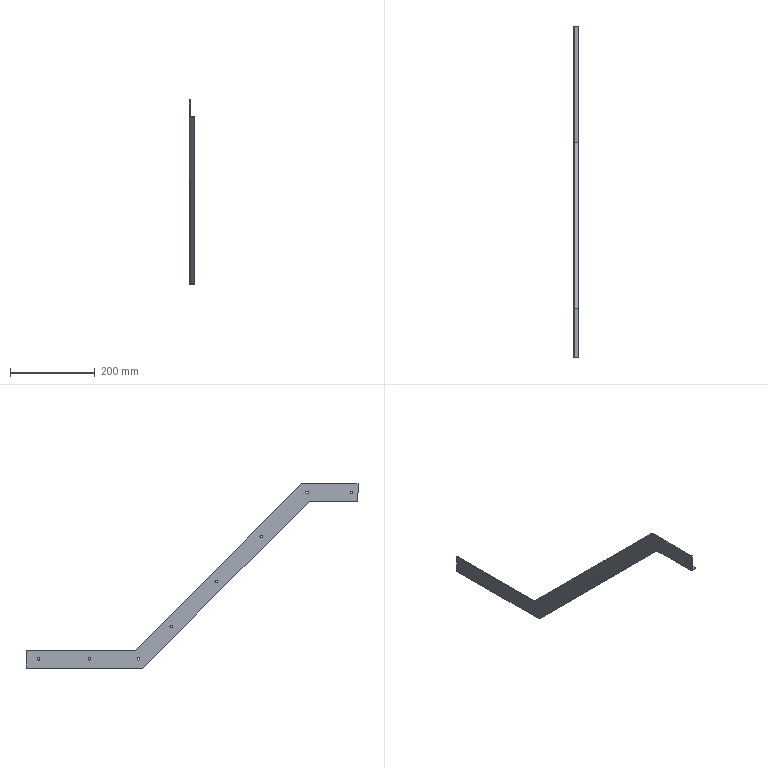Component | SolidWorks | ScraperPlate-1 | 1 solid | 30 faces | box 13 x 782.44 x 434.44 mm | volume 99718 mm3 | cylinder 16 | plane 14 | commonest cylinder face diameters 6 x16
build123d program:
from build123d import *

# Parameters (mm, degrees)
EXTRUDE_THIN1_DEPTH = 13
EXTRUDE_THIN2_DEPTH = 2
SKETCH4_R           = 3
CUT_EXTRUDE1_DEPTH  = 10


with BuildPart() as part:
    # Sketch1 → Extrude-Thin1 (new body)
    with BuildSketch(Plane.XY):
        Polygon((365.38, 490.188), (365.38, 215.188), (-27.064, -177.256), (-27.064, -292.256), (-29.064, -292.256), (-29.064, -176.427), (363.38, 216.017), (363.38, 490.188), align=None)
    extrude(amount=EXTRUDE_THIN1_DEPTH)

    # Sketch2 → Extrude-Thin2 (add)
    with BuildSketch(Plane(origin=(0, 0, 0), x_dir=(-1, 0, 0), z_dir=(0, 0, -1))):
        Polygon((-365.38, 490.188), (-365.38, 215.188), (27.064, -177.256), (27.064, -292.256), (69.064, -292.256), (69.064, -159.859), (-323.38, 232.585), (-323.38, 490.188), align=None)
    extrude(amount=-EXTRUDE_THIN2_DEPTH)

    # Sketch4 → Cut-Extrude1 (cut)
    with BuildSketch(Plane.XY.offset(2)):
        with Locations((343.38, 460.188)):
            Circle(SKETCH4_R)
        with Locations((343.38, 340.188)):
            Circle(SKETCH4_R)
        with Locations((267.057, 147.979)):
            Circle(SKETCH4_R)
        with Locations((160.991, 41.913)):
            Circle(SKETCH4_R)
        with Locations((54.925, -64.153)):
            Circle(SKETCH4_R)
        with Locations((-49.064, -277.256)):
            Circle(SKETCH4_R)
        with Locations((-49.064, -172.256)):
            Circle(SKETCH4_R)
        with Locations((343.38, 225.188)):
            Circle(SKETCH4_R)
    extrude(amount=-CUT_EXTRUDE1_DEPTH, mode=Mode.SUBTRACT)


solid = part.part

# Placed as in the assembly
solid = solid.moved(Location((-292.55, -121.313, -21.856), (0, 90, 0)))
STEP:
#1=CARTESIAN_POINT('',(-11.518,4.09,-14.497));
#2=VERTEX_POINT('',#1);
#3=CARTESIAN_POINT('',(-11.518,4.09,-14.261));
#4=VERTEX_POINT('',#3);
#5=CARTESIAN_POINT('',(-11.518,4.09,-14.379));
#6=DIRECTION('',(-1.,-0.,-0.));
#7=DIRECTION('',(0.,-0.,1.));
#8=AXIS2_PLACEMENT_3D('',#5,#6,#7);
#9=CIRCLE('',#8,0.1181);
#10=EDGE_CURVE('',#2,#4,#9,.T.);
#11=ORIENTED_EDGE('',*,*,#10,.T.);
#12=CARTESIAN_POINT('',(-11.439,4.09,-14.261));
#13=VERTEX_POINT('',#12);
#14=CARTESIAN_POINT('',(-11.833,4.09,-14.261));
#15=DIRECTION('',(1.,0.,0.));
#16=VECTOR('',#15,39.37);
#17=LINE('',#14,#16);
#18=EDGE_CURVE('',#4,#13,#17,.T.);
#19=ORIENTED_EDGE('',*,*,#18,.T.);
#20=CARTESIAN_POINT('',(-11.439,4.09,-14.497));
#21=VERTEX_POINT('',#20);
#22=CARTESIAN_POINT('',(-11.439,4.09,-14.379));
#23=DIRECTION('',(1.,0.,0.));
#24=DIRECTION('',(0.,0.,-1.));
#25=AXIS2_PLACEMENT_3D('',#22,#23,#24);
#26=CIRCLE('',#25,0.1181);
#27=EDGE_CURVE('',#13,#21,#26,.T.);
#28=ORIENTED_EDGE('',*,*,#27,.T.);
#29=CARTESIAN_POINT('',(-11.833,4.09,-14.497));
#30=DIRECTION('',(1.,0.,0.));
#31=VECTOR('',#30,39.37);
#32=LINE('',#29,#31);
#33=EDGE_CURVE('',#2,#21,#32,.T.);
#34=ORIENTED_EDGE('',*,*,#33,.F.);
#35=EDGE_LOOP('',(#11,#19,#28,#34));
#36=FACE_OUTER_BOUND('',#35,.T.);
#37=CARTESIAN_POINT('',(-11.833,4.09,-14.379));
#38=DIRECTION('',(1.,0.,0.));
#39=DIRECTION('',(0.,0.,-1.));
#40=AXIS2_PLACEMENT_3D('',#37,#38,#39);
#41=CYLINDRICAL_SURFACE('',#40,0.1181);
#42=ADVANCED_FACE('',(#36),#41,.F.);
#43=CARTESIAN_POINT('',(-11.518,-11.558,0.9531));
#44=VERTEX_POINT('',#43);
#45=CARTESIAN_POINT('',(-11.518,-11.558,1.189));
#46=VERTEX_POINT('',#45);
#47=CARTESIAN_POINT('',(-11.518,-11.558,1.071));
#48=DIRECTION('',(-1.,-0.,-0.));
#49=DIRECTION('',(0.,0.,1.));
#50=AXIS2_PLACEMENT_3D('',#47,#48,#49);
#51=CIRCLE('',#50,0.1181);
#52=EDGE_CURVE('',#44,#46,#51,.T.);
#53=ORIENTED_EDGE('',*,*,#52,.T.);
#54=CARTESIAN_POINT('',(-11.439,-11.558,1.189));
#55=VERTEX_POINT('',#54);
#56=CARTESIAN_POINT('',(-11.833,-11.558,1.189));
#57=DIRECTION('',(1.,0.,0.));
#58=VECTOR('',#57,39.37);
#59=LINE('',#56,#58);
#60=EDGE_CURVE('',#46,#55,#59,.T.);
#61=ORIENTED_EDGE('',*,*,#60,.T.);
#62=CARTESIAN_POINT('',(-11.439,-11.558,0.9531));
#63=VERTEX_POINT('',#62);
#64=CARTESIAN_POINT('',(-11.439,-11.558,1.071));
#65=DIRECTION('',(1.,0.,0.));
#66=DIRECTION('',(0.,0.,-1.));
#67=AXIS2_PLACEMENT_3D('',#64,#65,#66);
#68=CIRCLE('',#67,0.1181);
#69=EDGE_CURVE('',#55,#63,#68,.T.);
#70=ORIENTED_EDGE('',*,*,#69,.T.);
#71=CARTESIAN_POINT('',(-11.833,-11.558,0.9531));
#72=DIRECTION('',(1.,0.,0.));
#73=VECTOR('',#72,39.37);
#74=LINE('',#71,#73);
#75=EDGE_CURVE('',#44,#63,#74,.T.);
#76=ORIENTED_EDGE('',*,*,#75,.F.);
#77=EDGE_LOOP('',(#53,#61,#70,#76));
#78=FACE_OUTER_BOUND('',#77,.T.);
#79=CARTESIAN_POINT('',(-11.833,-11.558,1.071));
#80=DIRECTION('',(1.,0.,0.));
#81=DIRECTION('',(0.,0.,-1.));
#82=AXIS2_PLACEMENT_3D('',#79,#80,#81);
#83=CYLINDRICAL_SURFACE('',#82,0.1181);
#84=ADVANCED_FACE('',(#78),#83,.F.);
#85=CARTESIAN_POINT('',(-11.518,-15.692,0.9531));
#86=VERTEX_POINT('',#85);
#87=CARTESIAN_POINT('',(-11.518,-15.692,1.189));
#88=VERTEX_POINT('',#87);
#89=CARTESIAN_POINT('',(-11.518,-15.692,1.071));
#90=DIRECTION('',(-1.,-0.,-0.));
#91=DIRECTION('',(0.,0.,1.));
#92=AXIS2_PLACEMENT_3D('',#89,#90,#91);
#93=CIRCLE('',#92,0.1181);
#94=EDGE_CURVE('',#86,#88,#93,.T.);
#95=ORIENTED_EDGE('',*,*,#94,.T.);
#96=CARTESIAN_POINT('',(-11.439,-15.692,1.189));
#97=VERTEX_POINT('',#96);
#98=CARTESIAN_POINT('',(-11.833,-15.692,1.189));
#99=DIRECTION('',(1.,0.,0.));
#100=VECTOR('',#99,39.37);
#101=LINE('',#98,#100);
#102=EDGE_CURVE('',#88,#97,#101,.T.);
#103=ORIENTED_EDGE('',*,*,#102,.T.);
#104=CARTESIAN_POINT('',(-11.439,-15.692,0.9531));
#105=VERTEX_POINT('',#104);
#106=CARTESIAN_POINT('',(-11.439,-15.692,1.071));
#107=DIRECTION('',(1.,0.,0.));
#108=DIRECTION('',(0.,0.,-1.));
#109=AXIS2_PLACEMENT_3D('',#106,#107,#108);
#110=CIRCLE('',#109,0.1181);
#111=EDGE_CURVE('',#97,#105,#110,.T.);
#112=ORIENTED_EDGE('',*,*,#111,.T.);
#113=CARTESIAN_POINT('',(-11.833,-15.692,0.9531));
#114=DIRECTION('',(1.,0.,0.));
#115=VECTOR('',#114,39.37);
#116=LINE('',#113,#115);
#117=EDGE_CURVE('',#86,#105,#116,.T.);
#118=ORIENTED_EDGE('',*,*,#117,.F.);
#119=EDGE_LOOP('',(#95,#103,#112,#118));
#120=FACE_OUTER_BOUND('',#119,.T.);
#121=CARTESIAN_POINT('',(-11.833,-15.692,1.071));
#122=DIRECTION('',(1.,0.,0.));
#123=DIRECTION('',(0.,0.,-1.));
#124=AXIS2_PLACEMENT_3D('',#121,#122,#123);
#125=CYLINDRICAL_SURFACE('',#124,0.1181);
#126=ADVANCED_FACE('',(#120),#125,.F.);
#127=CARTESIAN_POINT('',(-11.518,-7.302,-3.141));
#128=VERTEX_POINT('',#127);
#129=CARTESIAN_POINT('',(-11.518,-7.302,-2.905));
#130=VERTEX_POINT('',#129);
#131=CARTESIAN_POINT('',(-11.518,-7.302,-3.023));
#132=DIRECTION('',(-1.,-0.,-0.));
#133=DIRECTION('',(0.,0.,1.));
#134=AXIS2_PLACEMENT_3D('',#131,#132,#133);
#135=CIRCLE('',#134,0.1181);
#136=EDGE_CURVE('',#128,#130,#135,.T.);
#137=ORIENTED_EDGE('',*,*,#136,.T.);
#138=CARTESIAN_POINT('',(-11.439,-7.302,-2.905));
#139=VERTEX_POINT('',#138);
#140=CARTESIAN_POINT('',(-11.833,-7.302,-2.905));
#141=DIRECTION('',(1.,0.,0.));
#142=VECTOR('',#141,39.37);
#143=LINE('',#140,#142);
#144=EDGE_CURVE('',#130,#139,#143,.T.);
#145=ORIENTED_EDGE('',*,*,#144,.T.);
#146=CARTESIAN_POINT('',(-11.439,-7.302,-3.141));
#147=VERTEX_POINT('',#146);
#148=CARTESIAN_POINT('',(-11.439,-7.302,-3.023));
#149=DIRECTION('',(1.,0.,0.));
#150=DIRECTION('',(0.,0.,-1.));
#151=AXIS2_PLACEMENT_3D('',#148,#149,#150);
#152=CIRCLE('',#151,0.1181);
#153=EDGE_CURVE('',#139,#147,#152,.T.);
#154=ORIENTED_EDGE('',*,*,#153,.T.);
#155=CARTESIAN_POINT('',(-11.833,-7.302,-3.141));
#156=DIRECTION('',(1.,0.,0.));
#157=VECTOR('',#156,39.37);
#158=LINE('',#155,#157);
#159=EDGE_CURVE('',#128,#147,#158,.T.);
#160=ORIENTED_EDGE('',*,*,#159,.F.);
#161=EDGE_LOOP('',(#137,#145,#154,#160));
#162=FACE_OUTER_BOUND('',#161,.T.);
#163=CARTESIAN_POINT('',(-11.833,-7.302,-3.023));
#164=DIRECTION('',(1.,0.,0.));
#165=DIRECTION('',(0.,0.,-1.));
#166=AXIS2_PLACEMENT_3D('',#163,#164,#165);
#167=CYLINDRICAL_SURFACE('',#166,0.1181);
#168=ADVANCED_FACE('',(#162),#167,.F.);
#169=CARTESIAN_POINT('',(-11.518,-3.126,-7.317));
#170=VERTEX_POINT('',#169);
#171=CARTESIAN_POINT('',(-11.518,-3.126,-7.081));
#172=VERTEX_POINT('',#171);
#173=CARTESIAN_POINT('',(-11.518,-3.126,-7.199));
#174=DIRECTION('',(-1.,-0.,-0.));
#175=DIRECTION('',(0.,-0.,1.));
#176=AXIS2_PLACEMENT_3D('',#173,#174,#175);
#177=CIRCLE('',#176,0.1181);
#178=EDGE_CURVE('',#170,#172,#177,.T.);
#179=ORIENTED_EDGE('',*,*,#178,.T.);
#180=CARTESIAN_POINT('',(-11.439,-3.126,-7.081));
#181=VERTEX_POINT('',#180);
#182=CARTESIAN_POINT('',(-11.833,-3.126,-7.081));
#183=DIRECTION('',(1.,0.,0.));
#184=VECTOR('',#183,39.37);
#185=LINE('',#182,#184);
#186=EDGE_CURVE('',#172,#181,#185,.T.);
#187=ORIENTED_EDGE('',*,*,#186,.T.);
#188=CARTESIAN_POINT('',(-11.439,-3.126,-7.317));
#189=VERTEX_POINT('',#188);
#190=CARTESIAN_POINT('',(-11.439,-3.126,-7.199));
#191=DIRECTION('',(1.,0.,0.));
#192=DIRECTION('',(0.,0.,-1.));
#193=AXIS2_PLACEMENT_3D('',#190,#191,#192);
#194=CIRCLE('',#193,0.1181);
#195=EDGE_CURVE('',#181,#189,#194,.T.);
#196=ORIENTED_EDGE('',*,*,#195,.T.);
#197=CARTESIAN_POINT('',(-11.833,-3.126,-7.317));
#198=DIRECTION('',(1.,0.,0.));
#199=VECTOR('',#198,39.37);
#200=LINE('',#197,#199);
#201=EDGE_CURVE('',#170,#189,#200,.T.);
#202=ORIENTED_EDGE('',*,*,#201,.F.);
#203=EDGE_LOOP('',(#179,#187,#196,#202));
#204=FACE_OUTER_BOUND('',#203,.T.);
#205=CARTESIAN_POINT('',(-11.833,-3.126,-7.199));
#206=DIRECTION('',(1.,0.,0.));
#207=DIRECTION('',(0.,0.,-1.));
#208=AXIS2_PLACEMENT_3D('',#205,#206,#207);
#209=CYLINDRICAL_SURFACE('',#208,0.1181);
#210=ADVANCED_FACE('',(#204),#209,.F.);
#211=CARTESIAN_POINT('',(-11.518,1.05,-11.493));
#212=VERTEX_POINT('',#211);
#213=CARTESIAN_POINT('',(-11.518,1.05,-11.256));
#214=VERTEX_POINT('',#213);
#215=CARTESIAN_POINT('',(-11.518,1.05,-11.375));
#216=DIRECTION('',(-1.,-0.,-0.));
#217=DIRECTION('',(0.,-0.,1.));
#218=AXIS2_PLACEMENT_3D('',#215,#216,#217);
#219=CIRCLE('',#218,0.1181);
#220=EDGE_CURVE('',#212,#214,#219,.T.);
#221=ORIENTED_EDGE('',*,*,#220,.T.);
#222=CARTESIAN_POINT('',(-11.439,1.05,-11.256));
#223=VERTEX_POINT('',#222);
#224=CARTESIAN_POINT('',(-11.833,1.05,-11.256));
#225=DIRECTION('',(1.,0.,0.));
#226=VECTOR('',#225,39.37);
#227=LINE('',#224,#226);
#228=EDGE_CURVE('',#214,#223,#227,.T.);
#229=ORIENTED_EDGE('',*,*,#228,.T.);
#230=CARTESIAN_POINT('',(-11.439,1.05,-11.493));
#231=VERTEX_POINT('',#230);
#232=CARTESIAN_POINT('',(-11.439,1.05,-11.375));
#233=DIRECTION('',(1.,0.,0.));
#234=DIRECTION('',(0.,0.,-1.));
#235=AXIS2_PLACEMENT_3D('',#232,#233,#234);
#236=CIRCLE('',#235,0.1181);
#237=EDGE_CURVE('',#223,#231,#236,.T.);
#238=ORIENTED_EDGE('',*,*,#237,.T.);
#239=CARTESIAN_POINT('',(-11.833,1.05,-11.493));
#240=DIRECTION('',(1.,0.,0.));
#241=VECTOR('',#240,39.37);
#242=LINE('',#239,#241);
#243=EDGE_CURVE('',#212,#231,#242,.T.);
#244=ORIENTED_EDGE('',*,*,#243,.F.);
#245=EDGE_LOOP('',(#221,#229,#238,#244));
#246=FACE_OUTER_BOUND('',#245,.T.);
#247=CARTESIAN_POINT('',(-11.833,1.05,-11.375));
#248=DIRECTION('',(1.,0.,0.));
#249=DIRECTION('',(0.,0.,-1.));
#250=AXIS2_PLACEMENT_3D('',#247,#248,#249);
#251=CYLINDRICAL_SURFACE('',#250,0.1181);
#252=ADVANCED_FACE('',(#246),#251,.F.);
#253=CARTESIAN_POINT('',(-11.518,8.617,-14.497));
#254=VERTEX_POINT('',#253);
#255=CARTESIAN_POINT('',(-11.518,8.617,-14.261));
#256=VERTEX_POINT('',#255);
#257=CARTESIAN_POINT('',(-11.518,8.617,-14.379));
#258=DIRECTION('',(-1.,-0.,-0.));
#259=DIRECTION('',(0.,0.,1.));
#260=AXIS2_PLACEMENT_3D('',#257,#258,#259);
#261=CIRCLE('',#260,0.1181);
#262=EDGE_CURVE('',#254,#256,#261,.T.);
#263=ORIENTED_EDGE('',*,*,#262,.T.);
#264=CARTESIAN_POINT('',(-11.439,8.617,-14.261));
#265=VERTEX_POINT('',#264);
#266=CARTESIAN_POINT('',(-11.833,8.617,-14.261));
#267=DIRECTION('',(1.,0.,0.));
#268=VECTOR('',#267,39.37);
#269=LINE('',#266,#268);
#270=EDGE_CURVE('',#256,#265,#269,.T.);
#271=ORIENTED_EDGE('',*,*,#270,.T.);
#272=CARTESIAN_POINT('',(-11.439,8.617,-14.497));
#273=VERTEX_POINT('',#272);
#274=CARTESIAN_POINT('',(-11.439,8.617,-14.379));
#275=DIRECTION('',(1.,0.,0.));
#276=DIRECTION('',(0.,0.,-1.));
#277=AXIS2_PLACEMENT_3D('',#274,#275,#276);
#278=CIRCLE('',#277,0.1181);
#279=EDGE_CURVE('',#265,#273,#278,.T.);
#280=ORIENTED_EDGE('',*,*,#279,.T.);
#281=CARTESIAN_POINT('',(-11.833,8.617,-14.497));
#282=DIRECTION('',(1.,0.,0.));
#283=VECTOR('',#282,39.37);
#284=LINE('',#281,#283);
#285=EDGE_CURVE('',#254,#273,#284,.T.);
#286=ORIENTED_EDGE('',*,*,#285,.F.);
#287=EDGE_LOOP('',(#263,#271,#280,#286));
#288=FACE_OUTER_BOUND('',#287,.T.);
#289=CARTESIAN_POINT('',(-11.833,8.617,-14.379));
#290=DIRECTION('',(1.,0.,0.));
#291=DIRECTION('',(0.,0.,-1.));
#292=AXIS2_PLACEMENT_3D('',#289,#290,#291);
#293=CYLINDRICAL_SURFACE('',#292,0.1181);
#294=ADVANCED_FACE('',(#288),#293,.F.);
#295=CARTESIAN_POINT('',(-11.518,13.342,-14.497));
#296=VERTEX_POINT('',#295);
#297=CARTESIAN_POINT('',(-11.518,13.342,-14.261));
#298=VERTEX_POINT('',#297);
#299=CARTESIAN_POINT('',(-11.518,13.342,-14.379));
#300=DIRECTION('',(-1.,-0.,-0.));
#301=DIRECTION('',(0.,0.,1.));
#302=AXIS2_PLACEMENT_3D('',#299,#300,#301);
#303=CIRCLE('',#302,0.1181);
#304=EDGE_CURVE('',#296,#298,#303,.T.);
#305=ORIENTED_EDGE('',*,*,#304,.T.);
#306=CARTESIAN_POINT('',(-11.439,13.342,-14.261));
#307=VERTEX_POINT('',#306);
#308=CARTESIAN_POINT('',(-11.833,13.342,-14.261));
#309=DIRECTION('',(1.,0.,0.));
#310=VECTOR('',#309,39.37);
#311=LINE('',#308,#310);
#312=EDGE_CURVE('',#298,#307,#311,.T.);
#313=ORIENTED_EDGE('',*,*,#312,.T.);
#314=CARTESIAN_POINT('',(-11.439,13.342,-14.497));
#315=VERTEX_POINT('',#314);
#316=CARTESIAN_POINT('',(-11.439,13.342,-14.379));
#317=DIRECTION('',(1.,0.,0.));
#318=DIRECTION('',(0.,0.,-1.));
#319=AXIS2_PLACEMENT_3D('',#316,#317,#318);
#320=CIRCLE('',#319,0.1181);
#321=EDGE_CURVE('',#307,#315,#320,.T.);
#322=ORIENTED_EDGE('',*,*,#321,.T.);
#323=CARTESIAN_POINT('',(-11.833,13.342,-14.497));
#324=DIRECTION('',(1.,0.,0.));
#325=VECTOR('',#324,39.37);
#326=LINE('',#323,#325);
#327=EDGE_CURVE('',#296,#315,#326,.T.);
#328=ORIENTED_EDGE('',*,*,#327,.F.);
#329=EDGE_LOOP('',(#305,#313,#322,#328));
#330=FACE_OUTER_BOUND('',#329,.T.);
#331=CARTESIAN_POINT('',(-11.833,13.342,-14.379));
#332=DIRECTION('',(1.,0.,0.));
#333=DIRECTION('',(0.,0.,-1.));
#334=AXIS2_PLACEMENT_3D('',#331,#332,#333);
#335=CYLINDRICAL_SURFACE('',#334,0.1181);
#336=ADVANCED_FACE('',(#330),#335,.F.);
#337=CARTESIAN_POINT('',(-11.006,-11.722,0.2838));
#338=VERTEX_POINT('',#337);
#339=CARTESIAN_POINT('',(-11.439,-11.722,0.2838));
#340=VERTEX_POINT('',#339);
#341=CARTESIAN_POINT('',(-11.006,-11.722,0.2838));
#342=DIRECTION('',(-1.,-0.,-0.));
#343=VECTOR('',#342,39.37);
#344=LINE('',#341,#343);
#345=EDGE_CURVE('',#338,#340,#344,.T.);
#346=ORIENTED_EDGE('',*,*,#345,.T.);
#347=CARTESIAN_POINT('',(-11.439,-16.282,0.2838));
#348=VERTEX_POINT('',#347);
#349=CARTESIAN_POINT('',(-11.439,-11.755,0.2838));
#350=DIRECTION('',(0.,-1.,-0.));
#351=VECTOR('',#350,39.37);
#352=LINE('',#349,#351);
#353=EDGE_CURVE('',#340,#348,#352,.T.);
#354=ORIENTED_EDGE('',*,*,#353,.T.);
#355=CARTESIAN_POINT('',(-11.006,-16.282,0.2838));
#356=VERTEX_POINT('',#355);
#357=CARTESIAN_POINT('',(-11.006,-16.282,0.2838));
#358=DIRECTION('',(-1.,-0.,-0.));
#359=VECTOR('',#358,39.37);
#360=LINE('',#357,#359);
#361=EDGE_CURVE('',#356,#348,#360,.T.);
#362=ORIENTED_EDGE('',*,*,#361,.F.);
#363=CARTESIAN_POINT('',(-11.006,-11.755,0.2838));
#364=DIRECTION('',(0.,-1.,-0.));
#365=VECTOR('',#364,39.37);
#366=LINE('',#363,#365);
#367=EDGE_CURVE('',#338,#356,#366,.T.);
#368=ORIENTED_EDGE('',*,*,#367,.F.);
#369=EDGE_LOOP('',(#346,#354,#362,#368));
#370=FACE_OUTER_BOUND('',#369,.T.);
#371=CARTESIAN_POINT('',(-11.006,-11.755,0.2838));
#372=DIRECTION('',(0.,0.,-1.));
#373=DIRECTION('',(-0.,1.,0.));
#374=AXIS2_PLACEMENT_3D('',#371,#372,#373);
#375=PLANE('',#374);
#376=ADVANCED_FACE('',(#370),#375,.F.);
#377=ORIENTED_EDGE('',*,*,#361,.T.);
#378=CARTESIAN_POINT('',(-11.439,-16.282,1.859));
#379=VERTEX_POINT('',#378);
#380=CARTESIAN_POINT('',(-11.439,-16.282,1.859));
#381=DIRECTION('',(0.,0.,-1.));
#382=VECTOR('',#381,39.37);
#383=LINE('',#380,#382);
#384=EDGE_CURVE('',#379,#348,#383,.T.);
#385=ORIENTED_EDGE('',*,*,#384,.F.);
#386=CARTESIAN_POINT('',(-11.518,-16.282,1.859));
#387=VERTEX_POINT('',#386);
#388=CARTESIAN_POINT('',(-11.439,-16.282,1.859));
#389=DIRECTION('',(-1.,-0.,-0.));
#390=VECTOR('',#389,39.37);
#391=LINE('',#388,#390);
#392=EDGE_CURVE('',#379,#387,#391,.T.);
#393=ORIENTED_EDGE('',*,*,#392,.T.);
#394=CARTESIAN_POINT('',(-11.518,-16.282,0.2051));
#395=VERTEX_POINT('',#394);
#396=CARTESIAN_POINT('',(-11.518,-16.282,0.2051));
#397=DIRECTION('',(-0.,-0.,1.));
#398=VECTOR('',#397,39.37);
#399=LINE('',#396,#398);
#400=EDGE_CURVE('',#395,#387,#399,.T.);
#401=ORIENTED_EDGE('',*,*,#400,.F.);
#402=CARTESIAN_POINT('',(-11.006,-16.282,0.2051));
#403=VERTEX_POINT('',#402);
#404=CARTESIAN_POINT('',(-11.006,-16.282,0.2051));
#405=DIRECTION('',(-1.,-0.,-0.));
#406=VECTOR('',#405,39.37);
#407=LINE('',#404,#406);
#408=EDGE_CURVE('',#403,#395,#407,.T.);
#409=ORIENTED_EDGE('',*,*,#408,.F.);
#410=CARTESIAN_POINT('',(-11.006,-16.282,0.2051));
#411=DIRECTION('',(-0.,-0.,1.));
#412=VECTOR('',#411,39.37);
#413=LINE('',#410,#412);
#414=EDGE_CURVE('',#403,#356,#413,.T.);
#415=ORIENTED_EDGE('',*,*,#414,.T.);
#416=EDGE_LOOP('',(#377,#385,#393,#401,#409,#415));
#417=FACE_OUTER_BOUND('',#416,.T.);
#418=CARTESIAN_POINT('',(-11.006,-16.282,0.2051));
#419=DIRECTION('',(0.,-1.,-0.));
#420=DIRECTION('',(-1.,-0.,-0.));
#421=AXIS2_PLACEMENT_3D('',#418,#419,#420);
#422=PLANE('',#421);
#423=ADVANCED_FACE('',(#417),#422,.T.);
#424=ORIENTED_EDGE('',*,*,#408,.T.);
#425=CARTESIAN_POINT('',(-11.518,-11.755,0.2051));
#426=VERTEX_POINT('',#425);
#427=CARTESIAN_POINT('',(-11.518,-11.755,0.2051));
#428=DIRECTION('',(0.,-1.,-0.));
#429=VECTOR('',#428,39.37);
#430=LINE('',#427,#429);
#431=EDGE_CURVE('',#426,#395,#430,.T.);
#432=ORIENTED_EDGE('',*,*,#431,.F.);
#433=CARTESIAN_POINT('',(-11.006,-11.755,0.2051));
#434=VERTEX_POINT('',#433);
#435=CARTESIAN_POINT('',(-11.006,-11.755,0.2051));
#436=DIRECTION('',(-1.,-0.,-0.));
#437=VECTOR('',#436,39.37);
#438=LINE('',#435,#437);
#439=EDGE_CURVE('',#434,#426,#438,.T.);
#440=ORIENTED_EDGE('',*,*,#439,.F.);
#441=CARTESIAN_POINT('',(-11.006,-11.755,0.2051));
#442=DIRECTION('',(0.,-1.,-0.));
#443=VECTOR('',#442,39.37);
#444=LINE('',#441,#443);
#445=EDGE_CURVE('',#434,#403,#444,.T.);
#446=ORIENTED_EDGE('',*,*,#445,.T.);
#447=EDGE_LOOP('',(#424,#432,#440,#446));
#448=FACE_OUTER_BOUND('',#447,.T.);
#449=CARTESIAN_POINT('',(-11.006,-11.755,0.2051));
#450=DIRECTION('',(0.,0.,-1.));
#451=DIRECTION('',(-0.,1.,0.));
#452=AXIS2_PLACEMENT_3D('',#449,#450,#451);
#453=PLANE('',#452);
#454=ADVANCED_FACE('',(#448),#453,.T.);
#455=ORIENTED_EDGE('',*,*,#439,.T.);
#456=CARTESIAN_POINT('',(-11.518,3.696,-15.245));
#457=VERTEX_POINT('',#456);
#458=CARTESIAN_POINT('',(-11.518,3.696,-15.245));
#459=DIRECTION('',(0.,-0.7071,0.7071));
#460=VECTOR('',#459,39.37);
#461=LINE('',#458,#460);
#462=EDGE_CURVE('',#457,#426,#461,.T.);
#463=ORIENTED_EDGE('',*,*,#462,.F.);
#464=CARTESIAN_POINT('',(-11.006,3.696,-15.245));
#465=VERTEX_POINT('',#464);
#466=CARTESIAN_POINT('',(-11.006,3.696,-15.245));
#467=DIRECTION('',(-1.,-0.,-0.));
#468=VECTOR('',#467,39.37);
#469=LINE('',#466,#468);
#470=EDGE_CURVE('',#465,#457,#469,.T.);
#471=ORIENTED_EDGE('',*,*,#470,.F.);
#472=CARTESIAN_POINT('',(-11.006,3.696,-15.245));
#473=DIRECTION('',(0.,-0.7071,0.7071));
#474=VECTOR('',#473,39.37);
#475=LINE('',#472,#474);
#476=EDGE_CURVE('',#465,#434,#475,.T.);
#477=ORIENTED_EDGE('',*,*,#476,.T.);
#478=EDGE_LOOP('',(#455,#463,#471,#477));
#479=FACE_OUTER_BOUND('',#478,.T.);
#480=CARTESIAN_POINT('',(-11.006,3.696,-15.245));
#481=DIRECTION('',(0.,-0.7071,-0.7071));
#482=DIRECTION('',(-0.,0.7071,-0.7071));
#483=AXIS2_PLACEMENT_3D('',#480,#481,#482);
#484=PLANE('',#483);
#485=ADVANCED_FACE('',(#479),#484,.T.);
#486=ORIENTED_EDGE('',*,*,#470,.T.);
#487=CARTESIAN_POINT('',(-11.518,14.523,-15.245));
#488=VERTEX_POINT('',#487);
#489=CARTESIAN_POINT('',(-11.518,14.523,-15.245));
#490=DIRECTION('',(0.,-1.,-0.));
#491=VECTOR('',#490,39.37);
#492=LINE('',#489,#491);
#493=EDGE_CURVE('',#488,#457,#492,.T.);
#494=ORIENTED_EDGE('',*,*,#493,.F.);
#495=CARTESIAN_POINT('',(-11.006,14.523,-15.245));
#496=VERTEX_POINT('',#495);
#497=CARTESIAN_POINT('',(-11.006,14.523,-15.245));
#498=DIRECTION('',(-1.,-0.,-0.));
#499=VECTOR('',#498,39.37);
#500=LINE('',#497,#499);
#501=EDGE_CURVE('',#496,#488,#500,.T.);
#502=ORIENTED_EDGE('',*,*,#501,.F.);
#503=CARTESIAN_POINT('',(-11.006,14.523,-15.245));
#504=DIRECTION('',(0.,-1.,-0.));
#505=VECTOR('',#504,39.37);
#506=LINE('',#503,#505);
#507=EDGE_CURVE('',#496,#465,#506,.T.);
#508=ORIENTED_EDGE('',*,*,#507,.T.);
#509=EDGE_LOOP('',(#486,#494,#502,#508));
#510=FACE_OUTER_BOUND('',#509,.T.);
#511=CARTESIAN_POINT('',(-11.006,14.523,-15.245));
#512=DIRECTION('',(0.,0.,-1.));
#513=DIRECTION('',(-1.,-0.,-0.));
#514=AXIS2_PLACEMENT_3D('',#511,#512,#513);
#515=PLANE('',#514);
#516=ADVANCED_FACE('',(#510),#515,.T.);
#517=ORIENTED_EDGE('',*,*,#501,.T.);
#518=CARTESIAN_POINT('',(-11.518,14.523,-13.592));
#519=VERTEX_POINT('',#518);
#520=CARTESIAN_POINT('',(-11.518,14.523,-15.167));
#521=DIRECTION('',(0.,0.,-1.));
#522=VECTOR('',#521,39.37);
#523=LINE('',#520,#522);
#524=EDGE_CURVE('',#519,#488,#523,.T.);
#525=ORIENTED_EDGE('',*,*,#524,.F.);
#526=CARTESIAN_POINT('',(-11.439,14.523,-13.592));
#527=VERTEX_POINT('',#526);
#528=CARTESIAN_POINT('',(-11.439,14.523,-13.592));
#529=DIRECTION('',(-1.,-0.,-0.));
#530=VECTOR('',#529,39.37);
#531=LINE('',#528,#530);
#532=EDGE_CURVE('',#527,#519,#531,.T.);
#533=ORIENTED_EDGE('',*,*,#532,.F.);
#534=CARTESIAN_POINT('',(-11.439,14.523,-15.167));
#535=VERTEX_POINT('',#534);
#536=CARTESIAN_POINT('',(-11.439,14.523,-15.245));
#537=DIRECTION('',(-0.,-0.,1.));
#538=VECTOR('',#537,39.37);
#539=LINE('',#536,#538);
#540=EDGE_CURVE('',#535,#527,#539,.T.);
#541=ORIENTED_EDGE('',*,*,#540,.F.);
#542=CARTESIAN_POINT('',(-11.006,14.523,-15.167));
#543=VERTEX_POINT('',#542);
#544=CARTESIAN_POINT('',(-11.006,14.523,-15.167));
#545=DIRECTION('',(-1.,-0.,-0.));
#546=VECTOR('',#545,39.37);
#547=LINE('',#544,#546);
#548=EDGE_CURVE('',#543,#535,#547,.T.);
#549=ORIENTED_EDGE('',*,*,#548,.F.);
#550=CARTESIAN_POINT('',(-11.006,14.523,-15.167));
#551=DIRECTION('',(0.,0.,-1.));
#552=VECTOR('',#551,39.37);
#553=LINE('',#550,#552);
#554=EDGE_CURVE('',#543,#496,#553,.T.);
#555=ORIENTED_EDGE('',*,*,#554,.T.);
#556=EDGE_LOOP('',(#517,#525,#533,#541,#549,#555));
#557=FACE_OUTER_BOUND('',#556,.T.);
#558=CARTESIAN_POINT('',(-11.006,14.523,-15.167));
#559=DIRECTION('',(-0.,1.,0.));
#560=DIRECTION('',(1.,0.,0.));
#561=AXIS2_PLACEMENT_3D('',#558,#559,#560);
#562=PLANE('',#561);
#563=ADVANCED_FACE('',(#557),#562,.T.);
#564=ORIENTED_EDGE('',*,*,#548,.T.);
#565=CARTESIAN_POINT('',(-11.439,3.729,-15.167));
#566=VERTEX_POINT('',#565);
#567=CARTESIAN_POINT('',(-11.439,14.523,-15.167));
#568=DIRECTION('',(0.,-1.,-0.));
#569=VECTOR('',#568,39.37);
#570=LINE('',#567,#569);
#571=EDGE_CURVE('',#535,#566,#570,.T.);
#572=ORIENTED_EDGE('',*,*,#571,.T.);
#573=CARTESIAN_POINT('',(-11.006,3.729,-15.167));
#574=VERTEX_POINT('',#573);
#575=CARTESIAN_POINT('',(-11.006,3.729,-15.167));
#576=DIRECTION('',(-1.,-0.,-0.));
#577=VECTOR('',#576,39.37);
#578=LINE('',#575,#577);
#579=EDGE_CURVE('',#574,#566,#578,.T.);
#580=ORIENTED_EDGE('',*,*,#579,.F.);
#581=CARTESIAN_POINT('',(-11.006,14.523,-15.167));
#582=DIRECTION('',(0.,-1.,-0.));
#583=VECTOR('',#582,39.37);
#584=LINE('',#581,#583);
#585=EDGE_CURVE('',#543,#574,#584,.T.);
#586=ORIENTED_EDGE('',*,*,#585,.F.);
#587=EDGE_LOOP('',(#564,#572,#580,#586));
#588=FACE_OUTER_BOUND('',#587,.T.);
#589=CARTESIAN_POINT('',(-11.006,14.523,-15.167));
#590=DIRECTION('',(0.,0.,-1.));
#591=DIRECTION('',(-1.,-0.,-0.));
#592=AXIS2_PLACEMENT_3D('',#589,#590,#591);
#593=PLANE('',#592);
#594=ADVANCED_FACE('',(#588),#593,.F.);
#595=ORIENTED_EDGE('',*,*,#579,.T.);
#596=CARTESIAN_POINT('',(-11.439,3.752,-15.19));
#597=DIRECTION('',(0.,-0.7071,0.7071));
#598=VECTOR('',#597,39.37);
#599=LINE('',#596,#598);
#600=EDGE_CURVE('',#566,#340,#599,.T.);
#601=ORIENTED_EDGE('',*,*,#600,.T.);
#602=ORIENTED_EDGE('',*,*,#345,.F.);
#603=CARTESIAN_POINT('',(-11.006,3.752,-15.19));
#604=DIRECTION('',(0.,-0.7071,0.7071));
#605=VECTOR('',#604,39.37);
#606=LINE('',#603,#605);
#607=EDGE_CURVE('',#574,#338,#606,.T.);
#608=ORIENTED_EDGE('',*,*,#607,.F.);
#609=EDGE_LOOP('',(#595,#601,#602,#608));
#610=FACE_OUTER_BOUND('',#609,.T.);
#611=CARTESIAN_POINT('',(-11.006,3.752,-15.19));
#612=DIRECTION('',(0.,-0.7071,-0.7071));
#613=DIRECTION('',(-0.,0.7071,-0.7071));
#614=AXIS2_PLACEMENT_3D('',#611,#612,#613);
#615=PLANE('',#614);
#616=ADVANCED_FACE('',(#610),#615,.F.);
#617=ORIENTED_EDGE('',*,*,#367,.T.);
#618=ORIENTED_EDGE('',*,*,#414,.F.);
#619=ORIENTED_EDGE('',*,*,#445,.F.);
#620=ORIENTED_EDGE('',*,*,#476,.F.);
#621=ORIENTED_EDGE('',*,*,#507,.F.);
#622=ORIENTED_EDGE('',*,*,#554,.F.);
#623=ORIENTED_EDGE('',*,*,#585,.T.);
#624=ORIENTED_EDGE('',*,*,#607,.T.);
#625=EDGE_LOOP('',(#617,#618,#619,#620,#621,#622,#623,#624));
#626=FACE_OUTER_BOUND('',#625,.T.);
#627=CARTESIAN_POINT('',(-11.006,-4.776,-0.8605));
#628=DIRECTION('',(-1.,-0.,-0.));
#629=DIRECTION('',(-0.,-0.,1.));
#630=AXIS2_PLACEMENT_3D('',#627,#628,#629);
#631=PLANE('',#630);
#632=ADVANCED_FACE('',(#626),#631,.F.);
#633=ORIENTED_EDGE('',*,*,#10,.F.);
#634=CARTESIAN_POINT('',(-11.518,4.09,-14.379));
#635=DIRECTION('',(-1.,-0.,-0.));
#636=DIRECTION('',(0.,-0.,1.));
#637=AXIS2_PLACEMENT_3D('',#634,#635,#636);
#638=CIRCLE('',#637,0.1181);
#639=EDGE_CURVE('',#4,#2,#638,.T.);
#640=ORIENTED_EDGE('',*,*,#639,.F.);
#641=EDGE_LOOP('',(#633,#640));
#642=FACE_BOUND('',#641,.T.);
#643=ORIENTED_EDGE('',*,*,#52,.F.);
#644=CARTESIAN_POINT('',(-11.518,-11.558,1.071));
#645=DIRECTION('',(-1.,-0.,-0.));
#646=DIRECTION('',(0.,0.,1.));
#647=AXIS2_PLACEMENT_3D('',#644,#645,#646);
#648=CIRCLE('',#647,0.1181);
#649=EDGE_CURVE('',#46,#44,#648,.T.);
#650=ORIENTED_EDGE('',*,*,#649,.F.);
#651=EDGE_LOOP('',(#643,#650));
#652=FACE_BOUND('',#651,.T.);
#653=ORIENTED_EDGE('',*,*,#94,.F.);
#654=CARTESIAN_POINT('',(-11.518,-15.692,1.071));
#655=DIRECTION('',(-1.,-0.,-0.));
#656=DIRECTION('',(0.,0.,1.));
#657=AXIS2_PLACEMENT_3D('',#654,#655,#656);
#658=CIRCLE('',#657,0.1181);
#659=EDGE_CURVE('',#88,#86,#658,.T.);
#660=ORIENTED_EDGE('',*,*,#659,.F.);
#661=EDGE_LOOP('',(#653,#660));
#662=FACE_BOUND('',#661,.T.);
#663=ORIENTED_EDGE('',*,*,#136,.F.);
#664=CARTESIAN_POINT('',(-11.518,-7.302,-3.023));
#665=DIRECTION('',(-1.,-0.,-0.));
#666=DIRECTION('',(0.,0.,1.));
#667=AXIS2_PLACEMENT_3D('',#664,#665,#666);
#668=CIRCLE('',#667,0.1181);
#669=EDGE_CURVE('',#130,#128,#668,.T.);
#670=ORIENTED_EDGE('',*,*,#669,.F.);
#671=EDGE_LOOP('',(#663,#670));
#672=FACE_BOUND('',#671,.T.);
#673=ORIENTED_EDGE('',*,*,#178,.F.);
#674=CARTESIAN_POINT('',(-11.518,-3.126,-7.199));
#675=DIRECTION('',(-1.,-0.,-0.));
#676=DIRECTION('',(0.,-0.,1.));
#677=AXIS2_PLACEMENT_3D('',#674,#675,#676);
#678=CIRCLE('',#677,0.1181);
#679=EDGE_CURVE('',#172,#170,#678,.T.);
#680=ORIENTED_EDGE('',*,*,#679,.F.);
#681=EDGE_LOOP('',(#673,#680));
#682=FACE_BOUND('',#681,.T.);
#683=ORIENTED_EDGE('',*,*,#220,.F.);
#684=CARTESIAN_POINT('',(-11.518,1.05,-11.375));
#685=DIRECTION('',(-1.,-0.,-0.));
#686=DIRECTION('',(0.,-0.,1.));
#687=AXIS2_PLACEMENT_3D('',#684,#685,#686);
#688=CIRCLE('',#687,0.1181);
#689=EDGE_CURVE('',#214,#212,#688,.T.);
#690=ORIENTED_EDGE('',*,*,#689,.F.);
#691=EDGE_LOOP('',(#683,#690));
#692=FACE_BOUND('',#691,.T.);
#693=ORIENTED_EDGE('',*,*,#262,.F.);
#694=CARTESIAN_POINT('',(-11.518,8.617,-14.379));
#695=DIRECTION('',(-1.,-0.,-0.));
#696=DIRECTION('',(0.,0.,1.));
#697=AXIS2_PLACEMENT_3D('',#694,#695,#696);
#698=CIRCLE('',#697,0.1181);
#699=EDGE_CURVE('',#256,#254,#698,.T.);
#700=ORIENTED_EDGE('',*,*,#699,.F.);
#701=EDGE_LOOP('',(#693,#700));
#702=FACE_BOUND('',#701,.T.);
#703=ORIENTED_EDGE('',*,*,#304,.F.);
#704=CARTESIAN_POINT('',(-11.518,13.342,-14.379));
#705=DIRECTION('',(-1.,-0.,-0.));
#706=DIRECTION('',(0.,0.,1.));
#707=AXIS2_PLACEMENT_3D('',#704,#705,#706);
#708=CIRCLE('',#707,0.1181);
#709=EDGE_CURVE('',#298,#296,#708,.T.);
#710=ORIENTED_EDGE('',*,*,#709,.F.);
#711=EDGE_LOOP('',(#703,#710));
#712=FACE_BOUND('',#711,.T.);
#713=ORIENTED_EDGE('',*,*,#400,.T.);
#714=CARTESIAN_POINT('',(-11.518,-11.07,1.859));
#715=VERTEX_POINT('',#714);
#716=CARTESIAN_POINT('',(-11.518,-11.755,1.859));
#717=DIRECTION('',(0.,-1.,-0.));
#718=VECTOR('',#717,39.37);
#719=LINE('',#716,#718);
#720=EDGE_CURVE('',#715,#387,#719,.T.);
#721=ORIENTED_EDGE('',*,*,#720,.F.);
#722=CARTESIAN_POINT('',(-11.518,4.381,-13.592));
#723=VERTEX_POINT('',#722);
#724=CARTESIAN_POINT('',(-11.518,4.865,-14.076));
#725=DIRECTION('',(0.,-0.7071,0.7071));
#726=VECTOR('',#725,39.37);
#727=LINE('',#724,#726);
#728=EDGE_CURVE('',#723,#715,#727,.T.);
#729=ORIENTED_EDGE('',*,*,#728,.F.);
#730=CARTESIAN_POINT('',(-11.518,14.523,-13.592));
#731=DIRECTION('',(0.,-1.,-0.));
#732=VECTOR('',#731,39.37);
#733=LINE('',#730,#732);
#734=EDGE_CURVE('',#519,#723,#733,.T.);
#735=ORIENTED_EDGE('',*,*,#734,.F.);
#736=ORIENTED_EDGE('',*,*,#524,.T.);
#737=ORIENTED_EDGE('',*,*,#493,.T.);
#738=ORIENTED_EDGE('',*,*,#462,.T.);
#739=ORIENTED_EDGE('',*,*,#431,.T.);
#740=EDGE_LOOP('',(#713,#721,#729,#735,#736,#737,#738,#739));
#741=FACE_OUTER_BOUND('',#740,.T.);
#742=CARTESIAN_POINT('',(-11.518,-4.776,-0.8605));
#743=DIRECTION('',(-1.,-0.,-0.));
#744=DIRECTION('',(-0.,-0.,1.));
#745=AXIS2_PLACEMENT_3D('',#742,#743,#744);
#746=PLANE('',#745);
#747=ADVANCED_FACE('',(#642,#652,#662,#672,#682,#692,#702,#712,#741),#746,.T.);
#748=CARTESIAN_POINT('',(-11.439,4.09,-14.379));
#749=DIRECTION('',(1.,0.,0.));
#750=DIRECTION('',(0.,0.,-1.));
#751=AXIS2_PLACEMENT_3D('',#748,#749,#750);
#752=CIRCLE('',#751,0.1181);
#753=EDGE_CURVE('',#21,#13,#752,.T.);
#754=ORIENTED_EDGE('',*,*,#753,.F.);
#755=ORIENTED_EDGE('',*,*,#27,.F.);
#756=EDGE_LOOP('',(#754,#755));
#757=FACE_BOUND('',#756,.T.);
#758=CARTESIAN_POINT('',(-11.439,-11.558,1.071));
#759=DIRECTION('',(1.,0.,0.));
#760=DIRECTION('',(0.,0.,-1.));
#761=AXIS2_PLACEMENT_3D('',#758,#759,#760);
#762=CIRCLE('',#761,0.1181);
#763=EDGE_CURVE('',#63,#55,#762,.T.);
#764=ORIENTED_EDGE('',*,*,#763,.F.);
#765=ORIENTED_EDGE('',*,*,#69,.F.);
#766=EDGE_LOOP('',(#764,#765));
#767=FACE_BOUND('',#766,.T.);
#768=CARTESIAN_POINT('',(-11.439,-15.692,1.071));
#769=DIRECTION('',(1.,0.,0.));
#770=DIRECTION('',(0.,0.,-1.));
#771=AXIS2_PLACEMENT_3D('',#768,#769,#770);
#772=CIRCLE('',#771,0.1181);
#773=EDGE_CURVE('',#105,#97,#772,.T.);
#774=ORIENTED_EDGE('',*,*,#773,.F.);
#775=ORIENTED_EDGE('',*,*,#111,.F.);
#776=EDGE_LOOP('',(#774,#775));
#777=FACE_BOUND('',#776,.T.);
#778=CARTESIAN_POINT('',(-11.439,-7.302,-3.023));
#779=DIRECTION('',(1.,0.,0.));
#780=DIRECTION('',(0.,0.,-1.));
#781=AXIS2_PLACEMENT_3D('',#778,#779,#780);
#782=CIRCLE('',#781,0.1181);
#783=EDGE_CURVE('',#147,#139,#782,.T.);
#784=ORIENTED_EDGE('',*,*,#783,.F.);
#785=ORIENTED_EDGE('',*,*,#153,.F.);
#786=EDGE_LOOP('',(#784,#785));
#787=FACE_BOUND('',#786,.T.);
#788=CARTESIAN_POINT('',(-11.439,-3.126,-7.199));
#789=DIRECTION('',(1.,0.,0.));
#790=DIRECTION('',(0.,0.,-1.));
#791=AXIS2_PLACEMENT_3D('',#788,#789,#790);
#792=CIRCLE('',#791,0.1181);
#793=EDGE_CURVE('',#189,#181,#792,.T.);
#794=ORIENTED_EDGE('',*,*,#793,.F.);
#795=ORIENTED_EDGE('',*,*,#195,.F.);
#796=EDGE_LOOP('',(#794,#795));
#797=FACE_BOUND('',#796,.T.);
#798=CARTESIAN_POINT('',(-11.439,1.05,-11.375));
#799=DIRECTION('',(1.,0.,0.));
#800=DIRECTION('',(0.,0.,-1.));
#801=AXIS2_PLACEMENT_3D('',#798,#799,#800);
#802=CIRCLE('',#801,0.1181);
#803=EDGE_CURVE('',#231,#223,#802,.T.);
#804=ORIENTED_EDGE('',*,*,#803,.F.);
#805=ORIENTED_EDGE('',*,*,#237,.F.);
#806=EDGE_LOOP('',(#804,#805));
#807=FACE_BOUND('',#806,.T.);
#808=CARTESIAN_POINT('',(-11.439,8.617,-14.379));
#809=DIRECTION('',(1.,0.,0.));
#810=DIRECTION('',(0.,0.,-1.));
#811=AXIS2_PLACEMENT_3D('',#808,#809,#810);
#812=CIRCLE('',#811,0.1181);
#813=EDGE_CURVE('',#273,#265,#812,.T.);
#814=ORIENTED_EDGE('',*,*,#813,.F.);
#815=ORIENTED_EDGE('',*,*,#279,.F.);
#816=EDGE_LOOP('',(#814,#815));
#817=FACE_BOUND('',#816,.T.);
#818=CARTESIAN_POINT('',(-11.439,13.342,-14.379));
#819=DIRECTION('',(1.,0.,0.));
#820=DIRECTION('',(0.,0.,-1.));
#821=AXIS2_PLACEMENT_3D('',#818,#819,#820);
#822=CIRCLE('',#821,0.1181);
#823=EDGE_CURVE('',#315,#307,#822,.T.);
#824=ORIENTED_EDGE('',*,*,#823,.F.);
#825=ORIENTED_EDGE('',*,*,#321,.F.);
#826=EDGE_LOOP('',(#824,#825));
#827=FACE_BOUND('',#826,.T.);
#828=ORIENTED_EDGE('',*,*,#353,.F.);
#829=ORIENTED_EDGE('',*,*,#600,.F.);
#830=ORIENTED_EDGE('',*,*,#571,.F.);
#831=ORIENTED_EDGE('',*,*,#540,.T.);
#832=CARTESIAN_POINT('',(-11.439,4.381,-13.592));
#833=VERTEX_POINT('',#832);
#834=CARTESIAN_POINT('',(-11.439,14.523,-13.592));
#835=DIRECTION('',(0.,-1.,-0.));
#836=VECTOR('',#835,39.37);
#837=LINE('',#834,#836);
#838=EDGE_CURVE('',#527,#833,#837,.T.);
#839=ORIENTED_EDGE('',*,*,#838,.T.);
#840=CARTESIAN_POINT('',(-11.439,-11.07,1.859));
#841=VERTEX_POINT('',#840);
#842=CARTESIAN_POINT('',(-11.439,4.865,-14.076));
#843=DIRECTION('',(0.,-0.7071,0.7071));
#844=VECTOR('',#843,39.37);
#845=LINE('',#842,#844);
#846=EDGE_CURVE('',#833,#841,#845,.T.);
#847=ORIENTED_EDGE('',*,*,#846,.T.);
#848=CARTESIAN_POINT('',(-11.439,-11.755,1.859));
#849=DIRECTION('',(0.,-1.,-0.));
#850=VECTOR('',#849,39.37);
#851=LINE('',#848,#850);
#852=EDGE_CURVE('',#841,#379,#851,.T.);
#853=ORIENTED_EDGE('',*,*,#852,.T.);
#854=ORIENTED_EDGE('',*,*,#384,.T.);
#855=EDGE_LOOP('',(#828,#829,#830,#831,#839,#847,#853,#854));
#856=FACE_OUTER_BOUND('',#855,.T.);
#857=CARTESIAN_POINT('',(-11.439,-4.776,-0.8605));
#858=DIRECTION('',(1.,0.,0.));
#859=DIRECTION('',(0.,0.,-1.));
#860=AXIS2_PLACEMENT_3D('',#857,#858,#859);
#861=PLANE('',#860);
#862=ADVANCED_FACE('',(#757,#767,#777,#787,#797,#807,#817,#827,#856),#861,.T.);
#863=ORIENTED_EDGE('',*,*,#734,.T.);
#864=CARTESIAN_POINT('',(-11.439,4.381,-13.592));
#865=DIRECTION('',(-1.,-0.,-0.));
#866=VECTOR('',#865,39.37);
#867=LINE('',#864,#866);
#868=EDGE_CURVE('',#833,#723,#867,.T.);
#869=ORIENTED_EDGE('',*,*,#868,.F.);
#870=ORIENTED_EDGE('',*,*,#838,.F.);
#871=ORIENTED_EDGE('',*,*,#532,.T.);
#872=EDGE_LOOP('',(#863,#869,#870,#871));
#873=FACE_OUTER_BOUND('',#872,.T.);
#874=CARTESIAN_POINT('',(-11.439,14.523,-13.592));
#875=DIRECTION('',(0.,0.,-1.));
#876=DIRECTION('',(-1.,-0.,-0.));
#877=AXIS2_PLACEMENT_3D('',#874,#875,#876);
#878=PLANE('',#877);
#879=ADVANCED_FACE('',(#873),#878,.F.);
#880=ORIENTED_EDGE('',*,*,#728,.T.);
#881=CARTESIAN_POINT('',(-11.439,-11.07,1.859));
#882=DIRECTION('',(-1.,-0.,-0.));
#883=VECTOR('',#882,39.37);
#884=LINE('',#881,#883);
#885=EDGE_CURVE('',#841,#715,#884,.T.);
#886=ORIENTED_EDGE('',*,*,#885,.F.);
#887=ORIENTED_EDGE('',*,*,#846,.F.);
#888=ORIENTED_EDGE('',*,*,#868,.T.);
#889=EDGE_LOOP('',(#880,#886,#887,#888));
#890=FACE_OUTER_BOUND('',#889,.T.);
#891=CARTESIAN_POINT('',(-11.439,4.865,-14.076));
#892=DIRECTION('',(0.,-0.7071,-0.7071));
#893=DIRECTION('',(-0.,0.7071,-0.7071));
#894=AXIS2_PLACEMENT_3D('',#891,#892,#893);
#895=PLANE('',#894);
#896=ADVANCED_FACE('',(#890),#895,.F.);
#897=ORIENTED_EDGE('',*,*,#720,.T.);
#898=ORIENTED_EDGE('',*,*,#392,.F.);
#899=ORIENTED_EDGE('',*,*,#852,.F.);
#900=ORIENTED_EDGE('',*,*,#885,.T.);
#901=EDGE_LOOP('',(#897,#898,#899,#900));
#902=FACE_OUTER_BOUND('',#901,.T.);
#903=CARTESIAN_POINT('',(-11.439,-11.755,1.859));
#904=DIRECTION('',(0.,0.,-1.));
#905=DIRECTION('',(-0.,1.,0.));
#906=AXIS2_PLACEMENT_3D('',#903,#904,#905);
#907=PLANE('',#906);
#908=ADVANCED_FACE('',(#902),#907,.F.);
#909=ORIENTED_EDGE('',*,*,#312,.F.);
#910=ORIENTED_EDGE('',*,*,#709,.T.);
#911=ORIENTED_EDGE('',*,*,#327,.T.);
#912=ORIENTED_EDGE('',*,*,#823,.T.);
#913=EDGE_LOOP('',(#909,#910,#911,#912));
#914=FACE_OUTER_BOUND('',#913,.T.);
#915=CARTESIAN_POINT('',(-11.833,13.342,-14.379));
#916=DIRECTION('',(1.,0.,0.));
#917=DIRECTION('',(0.,0.,-1.));
#918=AXIS2_PLACEMENT_3D('',#915,#916,#917);
#919=CYLINDRICAL_SURFACE('',#918,0.1181);
#920=ADVANCED_FACE('',(#914),#919,.F.);
#921=ORIENTED_EDGE('',*,*,#270,.F.);
#922=ORIENTED_EDGE('',*,*,#699,.T.);
#923=ORIENTED_EDGE('',*,*,#285,.T.);
#924=ORIENTED_EDGE('',*,*,#813,.T.);
#925=EDGE_LOOP('',(#921,#922,#923,#924));
#926=FACE_OUTER_BOUND('',#925,.T.);
#927=CARTESIAN_POINT('',(-11.833,8.617,-14.379));
#928=DIRECTION('',(1.,0.,0.));
#929=DIRECTION('',(0.,0.,-1.));
#930=AXIS2_PLACEMENT_3D('',#927,#928,#929);
#931=CYLINDRICAL_SURFACE('',#930,0.1181);
#932=ADVANCED_FACE('',(#926),#931,.F.);
#933=ORIENTED_EDGE('',*,*,#228,.F.);
#934=ORIENTED_EDGE('',*,*,#689,.T.);
#935=ORIENTED_EDGE('',*,*,#243,.T.);
#936=ORIENTED_EDGE('',*,*,#803,.T.);
#937=EDGE_LOOP('',(#933,#934,#935,#936));
#938=FACE_OUTER_BOUND('',#937,.T.);
#939=CARTESIAN_POINT('',(-11.833,1.05,-11.375));
#940=DIRECTION('',(1.,0.,0.));
#941=DIRECTION('',(0.,0.,-1.));
#942=AXIS2_PLACEMENT_3D('',#939,#940,#941);
#943=CYLINDRICAL_SURFACE('',#942,0.1181);
#944=ADVANCED_FACE('',(#938),#943,.F.);
#945=ORIENTED_EDGE('',*,*,#186,.F.);
#946=ORIENTED_EDGE('',*,*,#679,.T.);
#947=ORIENTED_EDGE('',*,*,#201,.T.);
#948=ORIENTED_EDGE('',*,*,#793,.T.);
#949=EDGE_LOOP('',(#945,#946,#947,#948));
#950=FACE_OUTER_BOUND('',#949,.T.);
#951=CARTESIAN_POINT('',(-11.833,-3.126,-7.199));
#952=DIRECTION('',(1.,0.,0.));
#953=DIRECTION('',(0.,0.,-1.));
#954=AXIS2_PLACEMENT_3D('',#951,#952,#953);
#955=CYLINDRICAL_SURFACE('',#954,0.1181);
#956=ADVANCED_FACE('',(#950),#955,.F.);
#957=ORIENTED_EDGE('',*,*,#144,.F.);
#958=ORIENTED_EDGE('',*,*,#669,.T.);
#959=ORIENTED_EDGE('',*,*,#159,.T.);
#960=ORIENTED_EDGE('',*,*,#783,.T.);
#961=EDGE_LOOP('',(#957,#958,#959,#960));
#962=FACE_OUTER_BOUND('',#961,.T.);
#963=CARTESIAN_POINT('',(-11.833,-7.302,-3.023));
#964=DIRECTION('',(1.,0.,0.));
#965=DIRECTION('',(0.,0.,-1.));
#966=AXIS2_PLACEMENT_3D('',#963,#964,#965);
#967=CYLINDRICAL_SURFACE('',#966,0.1181);
#968=ADVANCED_FACE('',(#962),#967,.F.);
#969=ORIENTED_EDGE('',*,*,#102,.F.);
#970=ORIENTED_EDGE('',*,*,#659,.T.);
#971=ORIENTED_EDGE('',*,*,#117,.T.);
#972=ORIENTED_EDGE('',*,*,#773,.T.);
#973=EDGE_LOOP('',(#969,#970,#971,#972));
#974=FACE_OUTER_BOUND('',#973,.T.);
#975=CARTESIAN_POINT('',(-11.833,-15.692,1.071));
#976=DIRECTION('',(1.,0.,0.));
#977=DIRECTION('',(0.,0.,-1.));
#978=AXIS2_PLACEMENT_3D('',#975,#976,#977);
#979=CYLINDRICAL_SURFACE('',#978,0.1181);
#980=ADVANCED_FACE('',(#974),#979,.F.);
#981=ORIENTED_EDGE('',*,*,#60,.F.);
#982=ORIENTED_EDGE('',*,*,#649,.T.);
#983=ORIENTED_EDGE('',*,*,#75,.T.);
#984=ORIENTED_EDGE('',*,*,#763,.T.);
#985=EDGE_LOOP('',(#981,#982,#983,#984));
#986=FACE_OUTER_BOUND('',#985,.T.);
#987=CARTESIAN_POINT('',(-11.833,-11.558,1.071));
#988=DIRECTION('',(1.,0.,0.));
#989=DIRECTION('',(0.,0.,-1.));
#990=AXIS2_PLACEMENT_3D('',#987,#988,#989);
#991=CYLINDRICAL_SURFACE('',#990,0.1181);
#992=ADVANCED_FACE('',(#986),#991,.F.);
#993=ORIENTED_EDGE('',*,*,#18,.F.);
#994=ORIENTED_EDGE('',*,*,#639,.T.);
#995=ORIENTED_EDGE('',*,*,#33,.T.);
#996=ORIENTED_EDGE('',*,*,#753,.T.);
#997=EDGE_LOOP('',(#993,#994,#995,#996));
#998=FACE_OUTER_BOUND('',#997,.T.);
#999=CARTESIAN_POINT('',(-11.833,4.09,-14.379));
#1000=DIRECTION('',(1.,0.,0.));
#1001=DIRECTION('',(0.,0.,-1.));
#1002=AXIS2_PLACEMENT_3D('',#999,#1000,#1001);
#1003=CYLINDRICAL_SURFACE('',#1002,0.1181);
#1004=ADVANCED_FACE('',(#998),#1003,.F.);
#1005=CLOSED_SHELL('',(#42,#84,#126,#168,#210,#252,#294,#336,#376,#423,#454,#485,#516,#563,#594,#616,#632,#747,#862,#879,#896,#908,#920,#932,#944,#956,#968,#980,#992,#1004));
#1006=MANIFOLD_SOLID_BREP('',#1005);
#1007=CARTESIAN_POINT('',(0.,0.,0.));
#1008=DIRECTION('',(0.,0.,1.));
#1009=DIRECTION('',(1.,0.,0.));
#1010=AXIS2_PLACEMENT_3D('',#1007,#1008,#1009);
#1011=(LENGTH_UNIT()NAMED_UNIT(*)SI_UNIT($,.METRE.));
#1012=LENGTH_MEASURE_WITH_UNIT(LENGTH_MEASURE(0.0254),#1011);
#1013=DIMENSIONAL_EXPONENTS(1.,0.,0.,0.,0.,0.,0.);
#1014=(CONVERSION_BASED_UNIT('',#1012)LENGTH_UNIT()NAMED_UNIT(#1013));
#1015=UNCERTAINTY_MEASURE_WITH_UNIT(LENGTH_MEASURE(0.00001),#1014,'','');
#1016=(NAMED_UNIT(*)PLANE_ANGLE_UNIT()SI_UNIT($,.RADIAN.));
#1017=(NAMED_UNIT(*)SI_UNIT($,.STERADIAN.)SOLID_ANGLE_UNIT());
#1018=(GEOMETRIC_REPRESENTATION_CONTEXT(3)GLOBAL_UNCERTAINTY_ASSIGNED_CONTEXT((#1015))GLOBAL_UNIT_ASSIGNED_CONTEXT((#1014,#1016,#1017))REPRESENTATION_CONTEXT('',''));
#1019=ADVANCED_BREP_SHAPE_REPRESENTATION('',(#1006,#1010),#1018);
#1020=COLOUR_RGB('',0.7922,0.8196,0.9333);
#1021=FILL_AREA_STYLE_COLOUR('',#1020);
#1022=FILL_AREA_STYLE('',(#1021));
#1023=SURFACE_STYLE_FILL_AREA(#1022);
#1024=SURFACE_SIDE_STYLE('',(#1023));
#1025=SURFACE_STYLE_USAGE(.BOTH.,#1024);
#1026=PRESENTATION_STYLE_ASSIGNMENT((#1025));
#1027=STYLED_ITEM('',(#1026),#1006);
#1028=(LENGTH_UNIT()NAMED_UNIT(*)SI_UNIT($,.METRE.));
#1029=LENGTH_MEASURE_WITH_UNIT(LENGTH_MEASURE(0.0254),#1028);
#1030=DIMENSIONAL_EXPONENTS(1.,0.,0.,0.,0.,0.,0.);
#1031=(CONVERSION_BASED_UNIT('',#1029)LENGTH_UNIT()NAMED_UNIT(#1030));
#1032=UNCERTAINTY_MEASURE_WITH_UNIT(LENGTH_MEASURE(0.00001),#1031,'','');
#1033=(NAMED_UNIT(*)PLANE_ANGLE_UNIT()SI_UNIT($,.RADIAN.));
#1034=(NAMED_UNIT(*)SI_UNIT($,.STERADIAN.)SOLID_ANGLE_UNIT());
#1035=(GEOMETRIC_REPRESENTATION_CONTEXT(3)GLOBAL_UNCERTAINTY_ASSIGNED_CONTEXT((#1032))GLOBAL_UNIT_ASSIGNED_CONTEXT((#1031,#1033,#1034))REPRESENTATION_CONTEXT('',''));
#1036=MECHANICAL_DESIGN_GEOMETRIC_PRESENTATION_REPRESENTATION('',(#1027),#1035);
#1037=PRESENTATION_LAYER_ASSIGNMENT('','',(#1027));